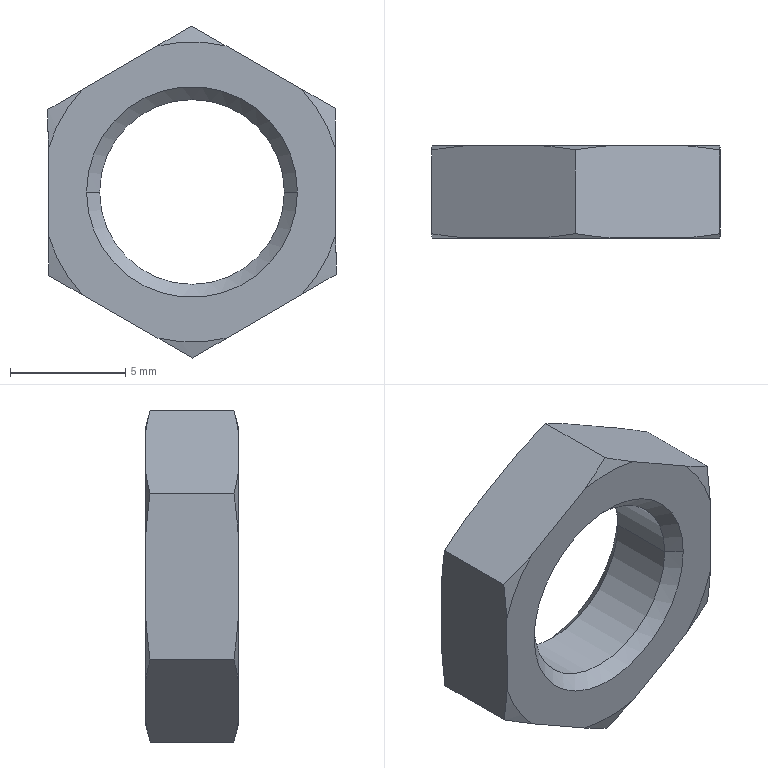Component | SolidWorks | GB_T6172.1-2000HexThinNutGradeAAndBM8-1 | 1 solid | 26 faces | box 12.48 x 4 x 14.38 mm | volume 327 mm3 | cone 16 | plane 8 | cylinder 2 | commonest cylinder face diameters 8 x2
STEP:
#1=COLOUR_RGB('',0.7922,0.8196,0.9333);
#2=FILL_AREA_STYLE_COLOUR('',#1);
#3=FILL_AREA_STYLE('',(#2));
#4=SURFACE_STYLE_FILL_AREA(#3);
#5=SURFACE_SIDE_STYLE('',(#4));
#6=SURFACE_STYLE_USAGE(.BOTH.,#5);
#7=PRESENTATION_STYLE_ASSIGNMENT((#6));
#8=CARTESIAN_POINT('',(2.795,-1.4,10.748));
#9=VERTEX_POINT('',#8);
#10=CARTESIAN_POINT('',(3.11,-1.4,10.748));
#11=VERTEX_POINT('',#10);
#12=CARTESIAN_POINT('',(2.953,-1.4,10.748));
#13=DIRECTION('',(0.,1.,0.));
#14=DIRECTION('',(-1.,0.,0.));
#15=AXIS2_PLACEMENT_3D('',#12,#13,#14);
#16=CIRCLE('',#15,0.1575);
#17=EDGE_CURVE('',#9,#11,#16,.T.);
#18=ORIENTED_EDGE('',*,*,#17,.F.);
#19=CARTESIAN_POINT('',(2.773,-1.378,10.748));
#20=VERTEX_POINT('',#19);
#21=CARTESIAN_POINT('',(2.795,-1.4,10.748));
#22=DIRECTION('',(-0.7071,0.7071,0.));
#23=VECTOR('',#22,39.37);
#24=LINE('',#21,#23);
#25=EDGE_CURVE('',#9,#20,#24,.T.);
#26=ORIENTED_EDGE('',*,*,#25,.T.);
#27=CARTESIAN_POINT('',(3.132,-1.378,10.748));
#28=VERTEX_POINT('',#27);
#29=CARTESIAN_POINT('',(2.953,-1.378,10.748));
#30=DIRECTION('',(0.,-1.,-0.));
#31=DIRECTION('',(-1.,0.,0.));
#32=AXIS2_PLACEMENT_3D('',#29,#30,#31);
#33=CIRCLE('',#32,0.1797);
#34=EDGE_CURVE('',#28,#20,#33,.T.);
#35=ORIENTED_EDGE('',*,*,#34,.F.);
#36=CARTESIAN_POINT('',(3.11,-1.4,10.748));
#37=DIRECTION('',(0.7071,0.7071,0.));
#38=VECTOR('',#37,39.37);
#39=LINE('',#36,#38);
#40=EDGE_CURVE('',#11,#28,#39,.T.);
#41=ORIENTED_EDGE('',*,*,#40,.F.);
#42=EDGE_LOOP('',(#18,#26,#35,#41));
#43=FACE_OUTER_BOUND('',#42,.T.);
#44=CARTESIAN_POINT('',(2.953,-1.4,10.748));
#45=DIRECTION('',(0.,1.,0.));
#46=DIRECTION('',(1.,0.,0.));
#47=AXIS2_PLACEMENT_3D('',#44,#45,#46);
#48=CONICAL_SURFACE('',#47,0.1575,0.7854);
#49=ADVANCED_FACE('',(#43),#48,.F.);
#50=CARTESIAN_POINT('',(3.11,-1.513,10.748));
#51=VERTEX_POINT('',#50);
#52=CARTESIAN_POINT('',(2.795,-1.513,10.748));
#53=VERTEX_POINT('',#52);
#54=CARTESIAN_POINT('',(2.953,-1.513,10.748));
#55=DIRECTION('',(0.,-1.,-0.));
#56=DIRECTION('',(-1.,0.,0.));
#57=AXIS2_PLACEMENT_3D('',#54,#55,#56);
#58=CIRCLE('',#57,0.1575);
#59=EDGE_CURVE('',#51,#53,#58,.T.);
#60=ORIENTED_EDGE('',*,*,#59,.F.);
#61=CARTESIAN_POINT('',(3.132,-1.535,10.748));
#62=VERTEX_POINT('',#61);
#63=CARTESIAN_POINT('',(3.132,-1.535,10.748));
#64=DIRECTION('',(0.7071,-0.7071,-0.));
#65=VECTOR('',#64,39.37);
#66=LINE('',#63,#65);
#67=EDGE_CURVE('',#51,#62,#66,.T.);
#68=ORIENTED_EDGE('',*,*,#67,.T.);
#69=CARTESIAN_POINT('',(2.773,-1.535,10.748));
#70=VERTEX_POINT('',#69);
#71=CARTESIAN_POINT('',(2.953,-1.535,10.748));
#72=DIRECTION('',(0.,1.,0.));
#73=DIRECTION('',(-1.,0.,0.));
#74=AXIS2_PLACEMENT_3D('',#71,#72,#73);
#75=CIRCLE('',#74,0.1797);
#76=EDGE_CURVE('',#70,#62,#75,.T.);
#77=ORIENTED_EDGE('',*,*,#76,.F.);
#78=CARTESIAN_POINT('',(2.773,-1.535,10.748));
#79=DIRECTION('',(-0.7071,-0.7071,-0.));
#80=VECTOR('',#79,39.37);
#81=LINE('',#78,#80);
#82=EDGE_CURVE('',#53,#70,#81,.T.);
#83=ORIENTED_EDGE('',*,*,#82,.F.);
#84=EDGE_LOOP('',(#60,#68,#77,#83));
#85=FACE_OUTER_BOUND('',#84,.T.);
#86=CARTESIAN_POINT('',(2.953,-1.535,10.748));
#87=DIRECTION('',(0.,-1.,-0.));
#88=DIRECTION('',(-1.,0.,0.));
#89=AXIS2_PLACEMENT_3D('',#86,#87,#88);
#90=CONICAL_SURFACE('',#89,0.1797,0.7854);
#91=ADVANCED_FACE('',(#85),#90,.F.);
#92=ORIENTED_EDGE('',*,*,#17,.T.);
#93=CARTESIAN_POINT('',(3.11,-1.378,10.748));
#94=DIRECTION('',(0.,-1.,-0.));
#95=VECTOR('',#94,39.37);
#96=LINE('',#93,#95);
#97=EDGE_CURVE('',#11,#51,#96,.T.);
#98=ORIENTED_EDGE('',*,*,#97,.T.);
#99=ORIENTED_EDGE('',*,*,#59,.T.);
#100=CARTESIAN_POINT('',(2.795,-1.378,10.748));
#101=DIRECTION('',(0.,-1.,-0.));
#102=VECTOR('',#101,39.37);
#103=LINE('',#100,#102);
#104=EDGE_CURVE('',#9,#53,#103,.T.);
#105=ORIENTED_EDGE('',*,*,#104,.F.);
#106=EDGE_LOOP('',(#92,#98,#99,#105));
#107=FACE_OUTER_BOUND('',#106,.T.);
#108=CARTESIAN_POINT('',(2.953,-1.378,10.748));
#109=DIRECTION('',(0.,-1.,-0.));
#110=DIRECTION('',(-1.,0.,0.));
#111=AXIS2_PLACEMENT_3D('',#108,#109,#110);
#112=CYLINDRICAL_SURFACE('',#111,0.1575);
#113=ADVANCED_FACE('',(#107),#112,.F.);
#114=CARTESIAN_POINT('',(2.767,-1.378,10.572));
#115=VERTEX_POINT('',#114);
#116=CARTESIAN_POINT('',(2.708,-1.385,10.606));
#117=VERTEX_POINT('',#116);
#118=CARTESIAN_POINT('',(2.767,-1.378,10.572));
#119=CARTESIAN_POINT('',(2.748,-1.38,10.583));
#120=CARTESIAN_POINT('',(2.728,-1.382,10.594));
#121=CARTESIAN_POINT('',(2.708,-1.385,10.606));
#122=B_SPLINE_CURVE_WITH_KNOTS('',3,(#118,#119,#120,#121),.UNSPECIFIED.,.F.,.F.,(4,4),(0.,0.00174),.UNSPECIFIED.);
#123=EDGE_CURVE('',#115,#117,#122,.T.);
#124=ORIENTED_EDGE('',*,*,#123,.T.);
#125=CARTESIAN_POINT('',(2.708,-1.378,10.674));
#126=VERTEX_POINT('',#125);
#127=CARTESIAN_POINT('',(2.708,-1.385,10.606));
#128=CARTESIAN_POINT('',(2.708,-1.382,10.628));
#129=CARTESIAN_POINT('',(2.708,-1.38,10.651));
#130=CARTESIAN_POINT('',(2.708,-1.378,10.674));
#131=B_SPLINE_CURVE_WITH_KNOTS('',3,(#127,#128,#129,#130),.UNSPECIFIED.,.F.,.F.,(4,4),(0.005002,0.006741),.UNSPECIFIED.);
#132=EDGE_CURVE('',#117,#126,#131,.T.);
#133=ORIENTED_EDGE('',*,*,#132,.T.);
#134=CARTESIAN_POINT('',(2.953,-1.378,10.748));
#135=DIRECTION('',(0.,-1.,-0.));
#136=DIRECTION('',(-1.,0.,0.));
#137=AXIS2_PLACEMENT_3D('',#134,#135,#136);
#138=CIRCLE('',#137,0.2559);
#139=EDGE_CURVE('',#126,#115,#138,.T.);
#140=ORIENTED_EDGE('',*,*,#139,.T.);
#141=EDGE_LOOP('',(#124,#133,#140));
#142=FACE_OUTER_BOUND('',#141,.T.);
#143=CARTESIAN_POINT('',(2.953,-1.378,10.748));
#144=DIRECTION('',(0.,-1.,-0.));
#145=DIRECTION('',(1.,0.,0.));
#146=AXIS2_PLACEMENT_3D('',#143,#144,#145);
#147=CONICAL_SURFACE('',#146,0.2559,1.309);
#148=ADVANCED_FACE('',(#142),#147,.T.);
#149=CARTESIAN_POINT('',(3.013,-1.378,10.499));
#150=VERTEX_POINT('',#149);
#151=CARTESIAN_POINT('',(2.954,-1.385,10.465));
#152=VERTEX_POINT('',#151);
#153=CARTESIAN_POINT('',(3.013,-1.378,10.499));
#154=CARTESIAN_POINT('',(2.993,-1.38,10.488));
#155=CARTESIAN_POINT('',(2.973,-1.382,10.476));
#156=CARTESIAN_POINT('',(2.954,-1.385,10.465));
#157=B_SPLINE_CURVE_WITH_KNOTS('',3,(#153,#154,#155,#156),.UNSPECIFIED.,.F.,.F.,(4,4),(0.,0.00174),.UNSPECIFIED.);
#158=EDGE_CURVE('',#150,#152,#157,.T.);
#159=ORIENTED_EDGE('',*,*,#158,.T.);
#160=CARTESIAN_POINT('',(2.895,-1.378,10.499));
#161=VERTEX_POINT('',#160);
#162=CARTESIAN_POINT('',(2.954,-1.385,10.465));
#163=CARTESIAN_POINT('',(2.934,-1.382,10.476));
#164=CARTESIAN_POINT('',(2.915,-1.38,10.487));
#165=CARTESIAN_POINT('',(2.895,-1.378,10.499));
#166=B_SPLINE_CURVE_WITH_KNOTS('',3,(#162,#163,#164,#165),.UNSPECIFIED.,.F.,.F.,(4,4),(0.00577,0.00751),.UNSPECIFIED.);
#167=EDGE_CURVE('',#152,#161,#166,.T.);
#168=ORIENTED_EDGE('',*,*,#167,.T.);
#169=CARTESIAN_POINT('',(2.953,-1.378,10.748));
#170=DIRECTION('',(0.,-1.,-0.));
#171=DIRECTION('',(-1.,0.,0.));
#172=AXIS2_PLACEMENT_3D('',#169,#170,#171);
#173=CIRCLE('',#172,0.2559);
#174=EDGE_CURVE('',#161,#150,#173,.T.);
#175=ORIENTED_EDGE('',*,*,#174,.T.);
#176=EDGE_LOOP('',(#159,#168,#175));
#177=FACE_OUTER_BOUND('',#176,.T.);
#178=CARTESIAN_POINT('',(2.953,-1.378,10.748));
#179=DIRECTION('',(0.,-1.,-0.));
#180=DIRECTION('',(1.,0.,0.));
#181=AXIS2_PLACEMENT_3D('',#178,#179,#180);
#182=CONICAL_SURFACE('',#181,0.2559,1.309);
#183=ADVANCED_FACE('',(#177),#182,.T.);
#184=CARTESIAN_POINT('',(3.198,-1.385,10.607));
#185=VERTEX_POINT('',#184);
#186=CARTESIAN_POINT('',(3.14,-1.378,10.573));
#187=VERTEX_POINT('',#186);
#188=CARTESIAN_POINT('',(3.198,-1.385,10.607));
#189=CARTESIAN_POINT('',(3.179,-1.382,10.596));
#190=CARTESIAN_POINT('',(3.159,-1.38,10.585));
#191=CARTESIAN_POINT('',(3.14,-1.378,10.573));
#192=B_SPLINE_CURVE_WITH_KNOTS('',3,(#188,#189,#190,#191),.UNSPECIFIED.,.F.,.F.,(4,4),(0.005796,0.007536),.UNSPECIFIED.);
#193=EDGE_CURVE('',#185,#187,#192,.T.);
#194=ORIENTED_EDGE('',*,*,#193,.T.);
#195=CARTESIAN_POINT('',(3.198,-1.378,10.676));
#196=VERTEX_POINT('',#195);
#197=CARTESIAN_POINT('',(2.953,-1.378,10.748));
#198=DIRECTION('',(0.,1.,0.));
#199=DIRECTION('',(1.,0.,0.));
#200=AXIS2_PLACEMENT_3D('',#197,#198,#199);
#201=CIRCLE('',#200,0.2559);
#202=EDGE_CURVE('',#196,#187,#201,.T.);
#203=ORIENTED_EDGE('',*,*,#202,.F.);
#204=CARTESIAN_POINT('',(3.198,-1.378,10.676));
#205=CARTESIAN_POINT('',(3.198,-1.38,10.653));
#206=CARTESIAN_POINT('',(3.198,-1.382,10.63));
#207=CARTESIAN_POINT('',(3.198,-1.385,10.607));
#208=B_SPLINE_CURVE_WITH_KNOTS('',3,(#204,#205,#206,#207),.UNSPECIFIED.,.F.,.F.,(4,4),(0.,0.00174),.UNSPECIFIED.);
#209=EDGE_CURVE('',#196,#185,#208,.T.);
#210=ORIENTED_EDGE('',*,*,#209,.T.);
#211=EDGE_LOOP('',(#194,#203,#210));
#212=FACE_OUTER_BOUND('',#211,.T.);
#213=CARTESIAN_POINT('',(2.953,-1.378,10.748));
#214=DIRECTION('',(0.,-1.,-0.));
#215=DIRECTION('',(1.,0.,0.));
#216=AXIS2_PLACEMENT_3D('',#213,#214,#215);
#217=CONICAL_SURFACE('',#216,0.2559,1.309);
#218=ADVANCED_FACE('',(#212),#217,.T.);
#219=CARTESIAN_POINT('',(3.138,-1.378,10.924));
#220=VERTEX_POINT('',#219);
#221=CARTESIAN_POINT('',(3.197,-1.385,10.891));
#222=VERTEX_POINT('',#221);
#223=CARTESIAN_POINT('',(3.138,-1.378,10.924));
#224=CARTESIAN_POINT('',(3.158,-1.38,10.913));
#225=CARTESIAN_POINT('',(3.178,-1.382,10.902));
#226=CARTESIAN_POINT('',(3.197,-1.385,10.891));
#227=B_SPLINE_CURVE_WITH_KNOTS('',3,(#223,#224,#225,#226),.UNSPECIFIED.,.F.,.F.,(4,4),(0.,0.00174),.UNSPECIFIED.);
#228=EDGE_CURVE('',#220,#222,#227,.T.);
#229=ORIENTED_EDGE('',*,*,#228,.T.);
#230=CARTESIAN_POINT('',(3.198,-1.378,10.822));
#231=VERTEX_POINT('',#230);
#232=CARTESIAN_POINT('',(3.197,-1.385,10.891));
#233=CARTESIAN_POINT('',(3.197,-1.382,10.868));
#234=CARTESIAN_POINT('',(3.198,-1.38,10.845));
#235=CARTESIAN_POINT('',(3.198,-1.378,10.822));
#236=B_SPLINE_CURVE_WITH_KNOTS('',3,(#232,#233,#234,#235),.UNSPECIFIED.,.F.,.F.,(4,4),(0.005002,0.006741),.UNSPECIFIED.);
#237=EDGE_CURVE('',#222,#231,#236,.T.);
#238=ORIENTED_EDGE('',*,*,#237,.T.);
#239=CARTESIAN_POINT('',(2.953,-1.378,10.748));
#240=DIRECTION('',(0.,-1.,-0.));
#241=DIRECTION('',(-1.,0.,0.));
#242=AXIS2_PLACEMENT_3D('',#239,#240,#241);
#243=CIRCLE('',#242,0.2559);
#244=EDGE_CURVE('',#231,#220,#243,.T.);
#245=ORIENTED_EDGE('',*,*,#244,.T.);
#246=EDGE_LOOP('',(#229,#238,#245));
#247=FACE_OUTER_BOUND('',#246,.T.);
#248=CARTESIAN_POINT('',(2.953,-1.378,10.748));
#249=DIRECTION('',(0.,-1.,-0.));
#250=DIRECTION('',(1.,0.,0.));
#251=AXIS2_PLACEMENT_3D('',#248,#249,#250);
#252=CONICAL_SURFACE('',#251,0.2559,1.309);
#253=ADVANCED_FACE('',(#247),#252,.T.);
#254=CARTESIAN_POINT('',(2.893,-1.378,10.997));
#255=VERTEX_POINT('',#254);
#256=CARTESIAN_POINT('',(2.952,-1.385,11.031));
#257=VERTEX_POINT('',#256);
#258=CARTESIAN_POINT('',(2.893,-1.378,10.997));
#259=CARTESIAN_POINT('',(2.912,-1.38,11.008));
#260=CARTESIAN_POINT('',(2.932,-1.382,11.02));
#261=CARTESIAN_POINT('',(2.952,-1.385,11.031));
#262=B_SPLINE_CURVE_WITH_KNOTS('',3,(#258,#259,#260,#261),.UNSPECIFIED.,.F.,.F.,(4,4),(0.,0.00174),.UNSPECIFIED.);
#263=EDGE_CURVE('',#255,#257,#262,.T.);
#264=ORIENTED_EDGE('',*,*,#263,.T.);
#265=CARTESIAN_POINT('',(3.011,-1.378,10.997));
#266=VERTEX_POINT('',#265);
#267=CARTESIAN_POINT('',(2.952,-1.385,11.031));
#268=CARTESIAN_POINT('',(2.971,-1.382,11.02));
#269=CARTESIAN_POINT('',(2.991,-1.38,11.009));
#270=CARTESIAN_POINT('',(3.011,-1.378,10.997));
#271=B_SPLINE_CURVE_WITH_KNOTS('',3,(#267,#268,#269,#270),.UNSPECIFIED.,.F.,.F.,(4,4),(0.00577,0.00751),.UNSPECIFIED.);
#272=EDGE_CURVE('',#257,#266,#271,.T.);
#273=ORIENTED_EDGE('',*,*,#272,.T.);
#274=CARTESIAN_POINT('',(2.953,-1.378,10.748));
#275=DIRECTION('',(0.,-1.,-0.));
#276=DIRECTION('',(-1.,0.,0.));
#277=AXIS2_PLACEMENT_3D('',#274,#275,#276);
#278=CIRCLE('',#277,0.2559);
#279=EDGE_CURVE('',#266,#255,#278,.T.);
#280=ORIENTED_EDGE('',*,*,#279,.T.);
#281=EDGE_LOOP('',(#264,#273,#280));
#282=FACE_OUTER_BOUND('',#281,.T.);
#283=CARTESIAN_POINT('',(2.953,-1.378,10.748));
#284=DIRECTION('',(0.,-1.,-0.));
#285=DIRECTION('',(1.,0.,0.));
#286=AXIS2_PLACEMENT_3D('',#283,#284,#285);
#287=CONICAL_SURFACE('',#286,0.2559,1.309);
#288=ADVANCED_FACE('',(#282),#287,.T.);
#289=CARTESIAN_POINT('',(2.707,-1.378,10.82));
#290=VERTEX_POINT('',#289);
#291=CARTESIAN_POINT('',(2.707,-1.385,10.889));
#292=VERTEX_POINT('',#291);
#293=CARTESIAN_POINT('',(2.707,-1.378,10.82));
#294=CARTESIAN_POINT('',(2.707,-1.38,10.843));
#295=CARTESIAN_POINT('',(2.707,-1.382,10.866));
#296=CARTESIAN_POINT('',(2.707,-1.385,10.889));
#297=B_SPLINE_CURVE_WITH_KNOTS('',3,(#293,#294,#295,#296),.UNSPECIFIED.,.F.,.F.,(4,4),(0.,0.00174),.UNSPECIFIED.);
#298=EDGE_CURVE('',#290,#292,#297,.T.);
#299=ORIENTED_EDGE('',*,*,#298,.T.);
#300=CARTESIAN_POINT('',(2.766,-1.378,10.923));
#301=VERTEX_POINT('',#300);
#302=CARTESIAN_POINT('',(2.707,-1.385,10.889));
#303=CARTESIAN_POINT('',(2.727,-1.382,10.9));
#304=CARTESIAN_POINT('',(2.746,-1.38,10.911));
#305=CARTESIAN_POINT('',(2.766,-1.378,10.923));
#306=B_SPLINE_CURVE_WITH_KNOTS('',3,(#302,#303,#304,#305),.UNSPECIFIED.,.F.,.F.,(4,4),(0.005796,0.007536),.UNSPECIFIED.);
#307=EDGE_CURVE('',#292,#301,#306,.T.);
#308=ORIENTED_EDGE('',*,*,#307,.T.);
#309=CARTESIAN_POINT('',(2.953,-1.378,10.748));
#310=DIRECTION('',(0.,-1.,-0.));
#311=DIRECTION('',(-1.,0.,0.));
#312=AXIS2_PLACEMENT_3D('',#309,#310,#311);
#313=CIRCLE('',#312,0.2559);
#314=EDGE_CURVE('',#301,#290,#313,.T.);
#315=ORIENTED_EDGE('',*,*,#314,.T.);
#316=EDGE_LOOP('',(#299,#308,#315));
#317=FACE_OUTER_BOUND('',#316,.T.);
#318=CARTESIAN_POINT('',(2.953,-1.378,10.748));
#319=DIRECTION('',(0.,-1.,-0.));
#320=DIRECTION('',(1.,0.,0.));
#321=AXIS2_PLACEMENT_3D('',#318,#319,#320);
#322=CONICAL_SURFACE('',#321,0.2559,1.309);
#323=ADVANCED_FACE('',(#317),#322,.T.);
#324=CARTESIAN_POINT('',(2.954,-1.528,10.465));
#325=VERTEX_POINT('',#324);
#326=CARTESIAN_POINT('',(3.013,-1.535,10.499));
#327=VERTEX_POINT('',#326);
#328=CARTESIAN_POINT('',(2.954,-1.528,10.465));
#329=CARTESIAN_POINT('',(2.973,-1.531,10.476));
#330=CARTESIAN_POINT('',(2.993,-1.534,10.488));
#331=CARTESIAN_POINT('',(3.013,-1.535,10.499));
#332=B_SPLINE_CURVE_WITH_KNOTS('',3,(#328,#329,#330,#331),.UNSPECIFIED.,.F.,.F.,(4,4),(0.005796,0.007536),.UNSPECIFIED.);
#333=EDGE_CURVE('',#325,#327,#332,.T.);
#334=ORIENTED_EDGE('',*,*,#333,.T.);
#335=CARTESIAN_POINT('',(2.895,-1.535,10.499));
#336=VERTEX_POINT('',#335);
#337=CARTESIAN_POINT('',(2.953,-1.535,10.748));
#338=DIRECTION('',(0.,-1.,-0.));
#339=DIRECTION('',(-1.,0.,0.));
#340=AXIS2_PLACEMENT_3D('',#337,#338,#339);
#341=CIRCLE('',#340,0.2559);
#342=EDGE_CURVE('',#336,#327,#341,.T.);
#343=ORIENTED_EDGE('',*,*,#342,.F.);
#344=CARTESIAN_POINT('',(2.895,-1.535,10.499));
#345=CARTESIAN_POINT('',(2.915,-1.534,10.487));
#346=CARTESIAN_POINT('',(2.934,-1.531,10.476));
#347=CARTESIAN_POINT('',(2.954,-1.528,10.465));
#348=B_SPLINE_CURVE_WITH_KNOTS('',3,(#344,#345,#346,#347),.UNSPECIFIED.,.F.,.F.,(4,4),(0.,0.00174),.UNSPECIFIED.);
#349=EDGE_CURVE('',#336,#325,#348,.T.);
#350=ORIENTED_EDGE('',*,*,#349,.T.);
#351=EDGE_LOOP('',(#334,#343,#350));
#352=FACE_OUTER_BOUND('',#351,.T.);
#353=CARTESIAN_POINT('',(2.953,-1.535,10.748));
#354=DIRECTION('',(0.,1.,0.));
#355=DIRECTION('',(-1.,0.,0.));
#356=AXIS2_PLACEMENT_3D('',#353,#354,#355);
#357=CONICAL_SURFACE('',#356,0.2559,1.309);
#358=ADVANCED_FACE('',(#352),#357,.T.);
#359=CARTESIAN_POINT('',(2.708,-1.528,10.606));
#360=VERTEX_POINT('',#359);
#361=CARTESIAN_POINT('',(2.767,-1.535,10.572));
#362=VERTEX_POINT('',#361);
#363=CARTESIAN_POINT('',(2.708,-1.528,10.606));
#364=CARTESIAN_POINT('',(2.728,-1.531,10.594));
#365=CARTESIAN_POINT('',(2.748,-1.534,10.583));
#366=CARTESIAN_POINT('',(2.767,-1.535,10.572));
#367=B_SPLINE_CURVE_WITH_KNOTS('',3,(#363,#364,#365,#366),.UNSPECIFIED.,.F.,.F.,(4,4),(0.00577,0.00751),.UNSPECIFIED.);
#368=EDGE_CURVE('',#360,#362,#367,.T.);
#369=ORIENTED_EDGE('',*,*,#368,.T.);
#370=CARTESIAN_POINT('',(2.708,-1.535,10.674));
#371=VERTEX_POINT('',#370);
#372=CARTESIAN_POINT('',(2.953,-1.535,10.748));
#373=DIRECTION('',(0.,-1.,-0.));
#374=DIRECTION('',(-1.,0.,0.));
#375=AXIS2_PLACEMENT_3D('',#372,#373,#374);
#376=CIRCLE('',#375,0.2559);
#377=EDGE_CURVE('',#371,#362,#376,.T.);
#378=ORIENTED_EDGE('',*,*,#377,.F.);
#379=CARTESIAN_POINT('',(2.708,-1.535,10.674));
#380=CARTESIAN_POINT('',(2.708,-1.534,10.651));
#381=CARTESIAN_POINT('',(2.708,-1.531,10.628));
#382=CARTESIAN_POINT('',(2.708,-1.528,10.606));
#383=B_SPLINE_CURVE_WITH_KNOTS('',3,(#379,#380,#381,#382),.UNSPECIFIED.,.F.,.F.,(4,4),(0.,0.00174),.UNSPECIFIED.);
#384=EDGE_CURVE('',#371,#360,#383,.T.);
#385=ORIENTED_EDGE('',*,*,#384,.T.);
#386=EDGE_LOOP('',(#369,#378,#385));
#387=FACE_OUTER_BOUND('',#386,.T.);
#388=CARTESIAN_POINT('',(2.953,-1.535,10.748));
#389=DIRECTION('',(0.,1.,0.));
#390=DIRECTION('',(-1.,0.,0.));
#391=AXIS2_PLACEMENT_3D('',#388,#389,#390);
#392=CONICAL_SURFACE('',#391,0.2559,1.309);
#393=ADVANCED_FACE('',(#387),#392,.T.);
#394=CARTESIAN_POINT('',(2.707,-1.528,10.889));
#395=VERTEX_POINT('',#394);
#396=CARTESIAN_POINT('',(2.707,-1.535,10.82));
#397=VERTEX_POINT('',#396);
#398=CARTESIAN_POINT('',(2.707,-1.528,10.889));
#399=CARTESIAN_POINT('',(2.707,-1.531,10.866));
#400=CARTESIAN_POINT('',(2.707,-1.534,10.843));
#401=CARTESIAN_POINT('',(2.707,-1.535,10.82));
#402=B_SPLINE_CURVE_WITH_KNOTS('',3,(#398,#399,#400,#401),.UNSPECIFIED.,.F.,.F.,(4,4),(0.005002,0.006741),.UNSPECIFIED.);
#403=EDGE_CURVE('',#395,#397,#402,.T.);
#404=ORIENTED_EDGE('',*,*,#403,.T.);
#405=CARTESIAN_POINT('',(2.766,-1.535,10.923));
#406=VERTEX_POINT('',#405);
#407=CARTESIAN_POINT('',(2.953,-1.535,10.748));
#408=DIRECTION('',(0.,-1.,-0.));
#409=DIRECTION('',(-1.,0.,0.));
#410=AXIS2_PLACEMENT_3D('',#407,#408,#409);
#411=CIRCLE('',#410,0.2559);
#412=EDGE_CURVE('',#406,#397,#411,.T.);
#413=ORIENTED_EDGE('',*,*,#412,.F.);
#414=CARTESIAN_POINT('',(2.766,-1.535,10.923));
#415=CARTESIAN_POINT('',(2.746,-1.534,10.911));
#416=CARTESIAN_POINT('',(2.727,-1.531,10.9));
#417=CARTESIAN_POINT('',(2.707,-1.528,10.889));
#418=B_SPLINE_CURVE_WITH_KNOTS('',3,(#414,#415,#416,#417),.UNSPECIFIED.,.F.,.F.,(4,4),(0.,0.00174),.UNSPECIFIED.);
#419=EDGE_CURVE('',#406,#395,#418,.T.);
#420=ORIENTED_EDGE('',*,*,#419,.T.);
#421=EDGE_LOOP('',(#404,#413,#420));
#422=FACE_OUTER_BOUND('',#421,.T.);
#423=CARTESIAN_POINT('',(2.953,-1.535,10.748));
#424=DIRECTION('',(0.,1.,0.));
#425=DIRECTION('',(-1.,0.,0.));
#426=AXIS2_PLACEMENT_3D('',#423,#424,#425);
#427=CONICAL_SURFACE('',#426,0.2559,1.309);
#428=ADVANCED_FACE('',(#422),#427,.T.);
#429=CARTESIAN_POINT('',(2.952,-1.528,11.031));
#430=VERTEX_POINT('',#429);
#431=CARTESIAN_POINT('',(2.893,-1.535,10.997));
#432=VERTEX_POINT('',#431);
#433=CARTESIAN_POINT('',(2.952,-1.528,11.031));
#434=CARTESIAN_POINT('',(2.932,-1.531,11.02));
#435=CARTESIAN_POINT('',(2.912,-1.534,11.008));
#436=CARTESIAN_POINT('',(2.893,-1.535,10.997));
#437=B_SPLINE_CURVE_WITH_KNOTS('',3,(#433,#434,#435,#436),.UNSPECIFIED.,.F.,.F.,(4,4),(0.005796,0.007536),.UNSPECIFIED.);
#438=EDGE_CURVE('',#430,#432,#437,.T.);
#439=ORIENTED_EDGE('',*,*,#438,.T.);
#440=CARTESIAN_POINT('',(3.011,-1.535,10.997));
#441=VERTEX_POINT('',#440);
#442=CARTESIAN_POINT('',(2.953,-1.535,10.748));
#443=DIRECTION('',(0.,-1.,-0.));
#444=DIRECTION('',(-1.,0.,0.));
#445=AXIS2_PLACEMENT_3D('',#442,#443,#444);
#446=CIRCLE('',#445,0.2559);
#447=EDGE_CURVE('',#441,#432,#446,.T.);
#448=ORIENTED_EDGE('',*,*,#447,.F.);
#449=CARTESIAN_POINT('',(3.011,-1.535,10.997));
#450=CARTESIAN_POINT('',(2.991,-1.534,11.009));
#451=CARTESIAN_POINT('',(2.971,-1.531,11.02));
#452=CARTESIAN_POINT('',(2.952,-1.528,11.031));
#453=B_SPLINE_CURVE_WITH_KNOTS('',3,(#449,#450,#451,#452),.UNSPECIFIED.,.F.,.F.,(4,4),(0.,0.00174),.UNSPECIFIED.);
#454=EDGE_CURVE('',#441,#430,#453,.T.);
#455=ORIENTED_EDGE('',*,*,#454,.T.);
#456=EDGE_LOOP('',(#439,#448,#455));
#457=FACE_OUTER_BOUND('',#456,.T.);
#458=CARTESIAN_POINT('',(2.953,-1.535,10.748));
#459=DIRECTION('',(0.,1.,0.));
#460=DIRECTION('',(-1.,0.,0.));
#461=AXIS2_PLACEMENT_3D('',#458,#459,#460);
#462=CONICAL_SURFACE('',#461,0.2559,1.309);
#463=ADVANCED_FACE('',(#457),#462,.T.);
#464=CARTESIAN_POINT('',(3.14,-1.535,10.573));
#465=VERTEX_POINT('',#464);
#466=CARTESIAN_POINT('',(3.198,-1.528,10.607));
#467=VERTEX_POINT('',#466);
#468=CARTESIAN_POINT('',(3.14,-1.535,10.573));
#469=CARTESIAN_POINT('',(3.159,-1.534,10.585));
#470=CARTESIAN_POINT('',(3.179,-1.531,10.596));
#471=CARTESIAN_POINT('',(3.198,-1.528,10.607));
#472=B_SPLINE_CURVE_WITH_KNOTS('',3,(#468,#469,#470,#471),.UNSPECIFIED.,.F.,.F.,(4,4),(0.,0.00174),.UNSPECIFIED.);
#473=EDGE_CURVE('',#465,#467,#472,.T.);
#474=ORIENTED_EDGE('',*,*,#473,.T.);
#475=CARTESIAN_POINT('',(3.198,-1.535,10.676));
#476=VERTEX_POINT('',#475);
#477=CARTESIAN_POINT('',(3.198,-1.528,10.607));
#478=CARTESIAN_POINT('',(3.198,-1.531,10.63));
#479=CARTESIAN_POINT('',(3.198,-1.534,10.653));
#480=CARTESIAN_POINT('',(3.198,-1.535,10.676));
#481=B_SPLINE_CURVE_WITH_KNOTS('',3,(#477,#478,#479,#480),.UNSPECIFIED.,.F.,.F.,(4,4),(0.005002,0.006741),.UNSPECIFIED.);
#482=EDGE_CURVE('',#467,#476,#481,.T.);
#483=ORIENTED_EDGE('',*,*,#482,.T.);
#484=CARTESIAN_POINT('',(2.953,-1.535,10.748));
#485=DIRECTION('',(0.,-1.,-0.));
#486=DIRECTION('',(-1.,0.,0.));
#487=AXIS2_PLACEMENT_3D('',#484,#485,#486);
#488=CIRCLE('',#487,0.2559);
#489=EDGE_CURVE('',#465,#476,#488,.T.);
#490=ORIENTED_EDGE('',*,*,#489,.F.);
#491=EDGE_LOOP('',(#474,#483,#490));
#492=FACE_OUTER_BOUND('',#491,.T.);
#493=CARTESIAN_POINT('',(2.953,-1.535,10.748));
#494=DIRECTION('',(0.,1.,0.));
#495=DIRECTION('',(-1.,0.,0.));
#496=AXIS2_PLACEMENT_3D('',#493,#494,#495);
#497=CONICAL_SURFACE('',#496,0.2559,1.309);
#498=ADVANCED_FACE('',(#492),#497,.T.);
#499=CARTESIAN_POINT('',(3.197,-1.528,10.891));
#500=VERTEX_POINT('',#499);
#501=CARTESIAN_POINT('',(3.138,-1.535,10.924));
#502=VERTEX_POINT('',#501);
#503=CARTESIAN_POINT('',(3.197,-1.528,10.891));
#504=CARTESIAN_POINT('',(3.178,-1.531,10.902));
#505=CARTESIAN_POINT('',(3.158,-1.534,10.913));
#506=CARTESIAN_POINT('',(3.138,-1.535,10.924));
#507=B_SPLINE_CURVE_WITH_KNOTS('',3,(#503,#504,#505,#506),.UNSPECIFIED.,.F.,.F.,(4,4),(0.00577,0.00751),.UNSPECIFIED.);
#508=EDGE_CURVE('',#500,#502,#507,.T.);
#509=ORIENTED_EDGE('',*,*,#508,.T.);
#510=CARTESIAN_POINT('',(3.198,-1.535,10.822));
#511=VERTEX_POINT('',#510);
#512=CARTESIAN_POINT('',(2.953,-1.535,10.748));
#513=DIRECTION('',(0.,-1.,-0.));
#514=DIRECTION('',(-1.,0.,0.));
#515=AXIS2_PLACEMENT_3D('',#512,#513,#514);
#516=CIRCLE('',#515,0.2559);
#517=EDGE_CURVE('',#511,#502,#516,.T.);
#518=ORIENTED_EDGE('',*,*,#517,.F.);
#519=CARTESIAN_POINT('',(3.198,-1.535,10.822));
#520=CARTESIAN_POINT('',(3.198,-1.534,10.845));
#521=CARTESIAN_POINT('',(3.197,-1.531,10.868));
#522=CARTESIAN_POINT('',(3.197,-1.528,10.891));
#523=B_SPLINE_CURVE_WITH_KNOTS('',3,(#519,#520,#521,#522),.UNSPECIFIED.,.F.,.F.,(4,4),(0.,0.00174),.UNSPECIFIED.);
#524=EDGE_CURVE('',#511,#500,#523,.T.);
#525=ORIENTED_EDGE('',*,*,#524,.T.);
#526=EDGE_LOOP('',(#509,#518,#525));
#527=FACE_OUTER_BOUND('',#526,.T.);
#528=CARTESIAN_POINT('',(2.953,-1.535,10.748));
#529=DIRECTION('',(0.,1.,0.));
#530=DIRECTION('',(-1.,0.,0.));
#531=AXIS2_PLACEMENT_3D('',#528,#529,#530);
#532=CONICAL_SURFACE('',#531,0.2559,1.309);
#533=ADVANCED_FACE('',(#527),#532,.T.);
#534=ORIENTED_EDGE('',*,*,#76,.T.);
#535=CARTESIAN_POINT('',(2.953,-1.535,10.748));
#536=DIRECTION('',(0.,1.,0.));
#537=DIRECTION('',(-1.,0.,0.));
#538=AXIS2_PLACEMENT_3D('',#535,#536,#537);
#539=CIRCLE('',#538,0.1797);
#540=EDGE_CURVE('',#62,#70,#539,.T.);
#541=ORIENTED_EDGE('',*,*,#540,.T.);
#542=EDGE_LOOP('',(#534,#541));
#543=FACE_BOUND('',#542,.T.);
#544=CARTESIAN_POINT('',(2.708,-1.535,10.606));
#545=DIRECTION('',(-0.003934,-0.,1.));
#546=VECTOR('',#545,39.37);
#547=LINE('',#544,#546);
#548=EDGE_CURVE('',#371,#397,#547,.T.);
#549=ORIENTED_EDGE('',*,*,#548,.F.);
#550=ORIENTED_EDGE('',*,*,#377,.T.);
#551=CARTESIAN_POINT('',(2.954,-1.535,10.465));
#552=DIRECTION('',(-0.868,-0.,0.4966));
#553=VECTOR('',#552,39.37);
#554=LINE('',#551,#553);
#555=EDGE_CURVE('',#336,#362,#554,.T.);
#556=ORIENTED_EDGE('',*,*,#555,.F.);
#557=ORIENTED_EDGE('',*,*,#342,.T.);
#558=CARTESIAN_POINT('',(3.198,-1.535,10.607));
#559=DIRECTION('',(-0.8641,0.,-0.5034));
#560=VECTOR('',#559,39.37);
#561=LINE('',#558,#560);
#562=EDGE_CURVE('',#465,#327,#561,.T.);
#563=ORIENTED_EDGE('',*,*,#562,.F.);
#564=ORIENTED_EDGE('',*,*,#489,.T.);
#565=CARTESIAN_POINT('',(3.197,-1.535,10.891));
#566=DIRECTION('',(0.003934,0.,-1.));
#567=VECTOR('',#566,39.37);
#568=LINE('',#565,#567);
#569=EDGE_CURVE('',#511,#476,#568,.T.);
#570=ORIENTED_EDGE('',*,*,#569,.F.);
#571=ORIENTED_EDGE('',*,*,#517,.T.);
#572=CARTESIAN_POINT('',(2.952,-1.535,11.031));
#573=DIRECTION('',(0.868,0.,-0.4966));
#574=VECTOR('',#573,39.37);
#575=LINE('',#572,#574);
#576=EDGE_CURVE('',#441,#502,#575,.T.);
#577=ORIENTED_EDGE('',*,*,#576,.F.);
#578=ORIENTED_EDGE('',*,*,#447,.T.);
#579=CARTESIAN_POINT('',(2.707,-1.535,10.889));
#580=DIRECTION('',(0.8641,-0.,0.5034));
#581=VECTOR('',#580,39.37);
#582=LINE('',#579,#581);
#583=EDGE_CURVE('',#406,#432,#582,.T.);
#584=ORIENTED_EDGE('',*,*,#583,.F.);
#585=ORIENTED_EDGE('',*,*,#412,.T.);
#586=EDGE_LOOP('',(#549,#550,#556,#557,#563,#564,#570,#571,#577,#578,#584,#585));
#587=FACE_OUTER_BOUND('',#586,.T.);
#588=CARTESIAN_POINT('',(3.443,-1.535,10.75));
#589=DIRECTION('',(0.,-1.,-0.));
#590=DIRECTION('',(0.,-0.,1.));
#591=AXIS2_PLACEMENT_3D('',#588,#589,#590);
#592=PLANE('',#591);
#593=ADVANCED_FACE('',(#543,#587),#592,.T.);
#594=ORIENTED_EDGE('',*,*,#34,.T.);
#595=CARTESIAN_POINT('',(2.953,-1.378,10.748));
#596=DIRECTION('',(0.,-1.,-0.));
#597=DIRECTION('',(-1.,0.,0.));
#598=AXIS2_PLACEMENT_3D('',#595,#596,#597);
#599=CIRCLE('',#598,0.1797);
#600=EDGE_CURVE('',#20,#28,#599,.T.);
#601=ORIENTED_EDGE('',*,*,#600,.T.);
#602=EDGE_LOOP('',(#594,#601));
#603=FACE_BOUND('',#602,.T.);
#604=ORIENTED_EDGE('',*,*,#139,.F.);
#605=CARTESIAN_POINT('',(2.708,-1.378,10.606));
#606=DIRECTION('',(-0.003934,-0.,1.));
#607=VECTOR('',#606,39.37);
#608=LINE('',#605,#607);
#609=EDGE_CURVE('',#126,#290,#608,.T.);
#610=ORIENTED_EDGE('',*,*,#609,.T.);
#611=ORIENTED_EDGE('',*,*,#314,.F.);
#612=CARTESIAN_POINT('',(2.707,-1.378,10.889));
#613=DIRECTION('',(0.8641,-0.,0.5034));
#614=VECTOR('',#613,39.37);
#615=LINE('',#612,#614);
#616=EDGE_CURVE('',#301,#255,#615,.T.);
#617=ORIENTED_EDGE('',*,*,#616,.T.);
#618=ORIENTED_EDGE('',*,*,#279,.F.);
#619=CARTESIAN_POINT('',(2.952,-1.378,11.031));
#620=DIRECTION('',(0.868,0.,-0.4966));
#621=VECTOR('',#620,39.37);
#622=LINE('',#619,#621);
#623=EDGE_CURVE('',#266,#220,#622,.T.);
#624=ORIENTED_EDGE('',*,*,#623,.T.);
#625=ORIENTED_EDGE('',*,*,#244,.F.);
#626=CARTESIAN_POINT('',(3.197,-1.378,10.891));
#627=DIRECTION('',(0.003934,0.,-1.));
#628=VECTOR('',#627,39.37);
#629=LINE('',#626,#628);
#630=EDGE_CURVE('',#231,#196,#629,.T.);
#631=ORIENTED_EDGE('',*,*,#630,.T.);
#632=ORIENTED_EDGE('',*,*,#202,.T.);
#633=CARTESIAN_POINT('',(3.198,-1.378,10.607));
#634=DIRECTION('',(-0.8641,0.,-0.5034));
#635=VECTOR('',#634,39.37);
#636=LINE('',#633,#635);
#637=EDGE_CURVE('',#187,#150,#636,.T.);
#638=ORIENTED_EDGE('',*,*,#637,.T.);
#639=ORIENTED_EDGE('',*,*,#174,.F.);
#640=CARTESIAN_POINT('',(2.954,-1.378,10.465));
#641=DIRECTION('',(-0.868,-0.,0.4966));
#642=VECTOR('',#641,39.37);
#643=LINE('',#640,#642);
#644=EDGE_CURVE('',#161,#115,#643,.T.);
#645=ORIENTED_EDGE('',*,*,#644,.T.);
#646=EDGE_LOOP('',(#604,#610,#611,#617,#618,#624,#625,#631,#632,#638,#639,#645));
#647=FACE_OUTER_BOUND('',#646,.T.);
#648=CARTESIAN_POINT('',(3.443,-1.378,10.75));
#649=DIRECTION('',(0.,-1.,-0.));
#650=DIRECTION('',(0.,-0.,1.));
#651=AXIS2_PLACEMENT_3D('',#648,#649,#650);
#652=PLANE('',#651);
#653=ADVANCED_FACE('',(#603,#647),#652,.F.);
#654=ORIENTED_EDGE('',*,*,#237,.F.);
#655=CARTESIAN_POINT('',(3.197,-1.378,10.891));
#656=DIRECTION('',(0.,-1.,-0.));
#657=VECTOR('',#656,39.37);
#658=LINE('',#655,#657);
#659=EDGE_CURVE('',#222,#500,#658,.T.);
#660=ORIENTED_EDGE('',*,*,#659,.T.);
#661=ORIENTED_EDGE('',*,*,#524,.F.);
#662=ORIENTED_EDGE('',*,*,#569,.T.);
#663=ORIENTED_EDGE('',*,*,#482,.F.);
#664=CARTESIAN_POINT('',(3.198,-1.378,10.607));
#665=DIRECTION('',(0.,-1.,-0.));
#666=VECTOR('',#665,39.37);
#667=LINE('',#664,#666);
#668=EDGE_CURVE('',#185,#467,#667,.T.);
#669=ORIENTED_EDGE('',*,*,#668,.F.);
#670=ORIENTED_EDGE('',*,*,#209,.F.);
#671=ORIENTED_EDGE('',*,*,#630,.F.);
#672=EDGE_LOOP('',(#654,#660,#661,#662,#663,#669,#670,#671));
#673=FACE_OUTER_BOUND('',#672,.T.);
#674=CARTESIAN_POINT('',(3.197,-1.378,10.891));
#675=DIRECTION('',(-1.,0.,-0.003934));
#676=DIRECTION('',(0.,1.,0.));
#677=AXIS2_PLACEMENT_3D('',#674,#675,#676);
#678=PLANE('',#677);
#679=ADVANCED_FACE('',(#673),#678,.F.);
#680=ORIENTED_EDGE('',*,*,#272,.F.);
#681=CARTESIAN_POINT('',(2.952,-1.378,11.031));
#682=DIRECTION('',(0.,-1.,-0.));
#683=VECTOR('',#682,39.37);
#684=LINE('',#681,#683);
#685=EDGE_CURVE('',#257,#430,#684,.T.);
#686=ORIENTED_EDGE('',*,*,#685,.T.);
#687=ORIENTED_EDGE('',*,*,#454,.F.);
#688=ORIENTED_EDGE('',*,*,#576,.T.);
#689=ORIENTED_EDGE('',*,*,#508,.F.);
#690=ORIENTED_EDGE('',*,*,#659,.F.);
#691=ORIENTED_EDGE('',*,*,#228,.F.);
#692=ORIENTED_EDGE('',*,*,#623,.F.);
#693=EDGE_LOOP('',(#680,#686,#687,#688,#689,#690,#691,#692));
#694=FACE_OUTER_BOUND('',#693,.T.);
#695=CARTESIAN_POINT('',(2.952,-1.378,11.031));
#696=DIRECTION('',(-0.4966,0.,-0.868));
#697=DIRECTION('',(0.,1.,0.));
#698=AXIS2_PLACEMENT_3D('',#695,#696,#697);
#699=PLANE('',#698);
#700=ADVANCED_FACE('',(#694),#699,.F.);
#701=ORIENTED_EDGE('',*,*,#307,.F.);
#702=CARTESIAN_POINT('',(2.707,-1.378,10.889));
#703=DIRECTION('',(0.,-1.,-0.));
#704=VECTOR('',#703,39.37);
#705=LINE('',#702,#704);
#706=EDGE_CURVE('',#292,#395,#705,.T.);
#707=ORIENTED_EDGE('',*,*,#706,.T.);
#708=ORIENTED_EDGE('',*,*,#419,.F.);
#709=ORIENTED_EDGE('',*,*,#583,.T.);
#710=ORIENTED_EDGE('',*,*,#438,.F.);
#711=ORIENTED_EDGE('',*,*,#685,.F.);
#712=ORIENTED_EDGE('',*,*,#263,.F.);
#713=ORIENTED_EDGE('',*,*,#616,.F.);
#714=EDGE_LOOP('',(#701,#707,#708,#709,#710,#711,#712,#713));
#715=FACE_OUTER_BOUND('',#714,.T.);
#716=CARTESIAN_POINT('',(2.707,-1.378,10.889));
#717=DIRECTION('',(0.5034,0.,-0.8641));
#718=DIRECTION('',(0.,-1.,-0.));
#719=AXIS2_PLACEMENT_3D('',#716,#717,#718);
#720=PLANE('',#719);
#721=ADVANCED_FACE('',(#715),#720,.F.);
#722=ORIENTED_EDGE('',*,*,#132,.F.);
#723=CARTESIAN_POINT('',(2.708,-1.378,10.606));
#724=DIRECTION('',(0.,-1.,-0.));
#725=VECTOR('',#724,39.37);
#726=LINE('',#723,#725);
#727=EDGE_CURVE('',#117,#360,#726,.T.);
#728=ORIENTED_EDGE('',*,*,#727,.T.);
#729=ORIENTED_EDGE('',*,*,#384,.F.);
#730=ORIENTED_EDGE('',*,*,#548,.T.);
#731=ORIENTED_EDGE('',*,*,#403,.F.);
#732=ORIENTED_EDGE('',*,*,#706,.F.);
#733=ORIENTED_EDGE('',*,*,#298,.F.);
#734=ORIENTED_EDGE('',*,*,#609,.F.);
#735=EDGE_LOOP('',(#722,#728,#729,#730,#731,#732,#733,#734));
#736=FACE_OUTER_BOUND('',#735,.T.);
#737=CARTESIAN_POINT('',(2.708,-1.378,10.606));
#738=DIRECTION('',(1.,-0.,0.003934));
#739=DIRECTION('',(0.,-1.,-0.));
#740=AXIS2_PLACEMENT_3D('',#737,#738,#739);
#741=PLANE('',#740);
#742=ADVANCED_FACE('',(#736),#741,.F.);
#743=ORIENTED_EDGE('',*,*,#167,.F.);
#744=CARTESIAN_POINT('',(2.954,-1.378,10.465));
#745=DIRECTION('',(0.,-1.,-0.));
#746=VECTOR('',#745,39.37);
#747=LINE('',#744,#746);
#748=EDGE_CURVE('',#152,#325,#747,.T.);
#749=ORIENTED_EDGE('',*,*,#748,.T.);
#750=ORIENTED_EDGE('',*,*,#349,.F.);
#751=ORIENTED_EDGE('',*,*,#555,.T.);
#752=ORIENTED_EDGE('',*,*,#368,.F.);
#753=ORIENTED_EDGE('',*,*,#727,.F.);
#754=ORIENTED_EDGE('',*,*,#123,.F.);
#755=ORIENTED_EDGE('',*,*,#644,.F.);
#756=EDGE_LOOP('',(#743,#749,#750,#751,#752,#753,#754,#755));
#757=FACE_OUTER_BOUND('',#756,.T.);
#758=CARTESIAN_POINT('',(2.954,-1.378,10.465));
#759=DIRECTION('',(0.4966,-0.,0.868));
#760=DIRECTION('',(0.,-1.,-0.));
#761=AXIS2_PLACEMENT_3D('',#758,#759,#760);
#762=PLANE('',#761);
#763=ADVANCED_FACE('',(#757),#762,.F.);
#764=ORIENTED_EDGE('',*,*,#193,.F.);
#765=ORIENTED_EDGE('',*,*,#668,.T.);
#766=ORIENTED_EDGE('',*,*,#473,.F.);
#767=ORIENTED_EDGE('',*,*,#562,.T.);
#768=ORIENTED_EDGE('',*,*,#333,.F.);
#769=ORIENTED_EDGE('',*,*,#748,.F.);
#770=ORIENTED_EDGE('',*,*,#158,.F.);
#771=ORIENTED_EDGE('',*,*,#637,.F.);
#772=EDGE_LOOP('',(#764,#765,#766,#767,#768,#769,#770,#771));
#773=FACE_OUTER_BOUND('',#772,.T.);
#774=CARTESIAN_POINT('',(3.198,-1.378,10.607));
#775=DIRECTION('',(-0.5034,-0.,0.8641));
#776=DIRECTION('',(-0.8641,0.,-0.5034));
#777=AXIS2_PLACEMENT_3D('',#774,#775,#776);
#778=PLANE('',#777);
#779=ADVANCED_FACE('',(#773),#778,.F.);
#780=ORIENTED_EDGE('',*,*,#97,.F.);
#781=CARTESIAN_POINT('',(2.953,-1.4,10.748));
#782=DIRECTION('',(0.,1.,0.));
#783=DIRECTION('',(-1.,0.,0.));
#784=AXIS2_PLACEMENT_3D('',#781,#782,#783);
#785=CIRCLE('',#784,0.1575);
#786=EDGE_CURVE('',#11,#9,#785,.T.);
#787=ORIENTED_EDGE('',*,*,#786,.T.);
#788=ORIENTED_EDGE('',*,*,#104,.T.);
#789=CARTESIAN_POINT('',(2.953,-1.513,10.748));
#790=DIRECTION('',(0.,-1.,-0.));
#791=DIRECTION('',(-1.,0.,0.));
#792=AXIS2_PLACEMENT_3D('',#789,#790,#791);
#793=CIRCLE('',#792,0.1575);
#794=EDGE_CURVE('',#53,#51,#793,.T.);
#795=ORIENTED_EDGE('',*,*,#794,.T.);
#796=EDGE_LOOP('',(#780,#787,#788,#795));
#797=FACE_OUTER_BOUND('',#796,.T.);
#798=CARTESIAN_POINT('',(2.953,-1.378,10.748));
#799=DIRECTION('',(0.,-1.,-0.));
#800=DIRECTION('',(-1.,0.,0.));
#801=AXIS2_PLACEMENT_3D('',#798,#799,#800);
#802=CYLINDRICAL_SURFACE('',#801,0.1575);
#803=ADVANCED_FACE('',(#797),#802,.F.);
#804=ORIENTED_EDGE('',*,*,#67,.F.);
#805=ORIENTED_EDGE('',*,*,#794,.F.);
#806=ORIENTED_EDGE('',*,*,#82,.T.);
#807=ORIENTED_EDGE('',*,*,#540,.F.);
#808=EDGE_LOOP('',(#804,#805,#806,#807));
#809=FACE_OUTER_BOUND('',#808,.T.);
#810=CARTESIAN_POINT('',(2.953,-1.535,10.748));
#811=DIRECTION('',(0.,-1.,-0.));
#812=DIRECTION('',(-1.,0.,0.));
#813=AXIS2_PLACEMENT_3D('',#810,#811,#812);
#814=CONICAL_SURFACE('',#813,0.1797,0.7854);
#815=ADVANCED_FACE('',(#809),#814,.F.);
#816=ORIENTED_EDGE('',*,*,#25,.F.);
#817=ORIENTED_EDGE('',*,*,#786,.F.);
#818=ORIENTED_EDGE('',*,*,#40,.T.);
#819=ORIENTED_EDGE('',*,*,#600,.F.);
#820=EDGE_LOOP('',(#816,#817,#818,#819));
#821=FACE_OUTER_BOUND('',#820,.T.);
#822=CARTESIAN_POINT('',(2.953,-1.4,10.748));
#823=DIRECTION('',(0.,1.,0.));
#824=DIRECTION('',(1.,0.,0.));
#825=AXIS2_PLACEMENT_3D('',#822,#823,#824);
#826=CONICAL_SURFACE('',#825,0.1575,0.7854);
#827=ADVANCED_FACE('',(#821),#826,.F.);
#828=CLOSED_SHELL('',(#49,#91,#113,#148,#183,#218,#253,#288,#323,#358,#393,#428,#463,#498,#533,#593,#653,#679,#700,#721,#742,#763,#779,#803,#815,#827));
#829=MANIFOLD_SOLID_BREP('',#828);
#830=STYLED_ITEM('',(#7),#829);
#831=PRESENTATION_LAYER_ASSIGNMENT('','',(#830));
#832=(LENGTH_UNIT()NAMED_UNIT(*)SI_UNIT($,.METRE.));
#833=LENGTH_MEASURE_WITH_UNIT(LENGTH_MEASURE(0.0254),#832);
#834=DIMENSIONAL_EXPONENTS(1.,0.,0.,0.,0.,0.,0.);
#835=(CONVERSION_BASED_UNIT('',#833)LENGTH_UNIT()NAMED_UNIT(#834));
#836=UNCERTAINTY_MEASURE_WITH_UNIT(LENGTH_MEASURE(0.00001),#835,'','');
#837=(NAMED_UNIT(*)PLANE_ANGLE_UNIT()SI_UNIT($,.RADIAN.));
#838=(NAMED_UNIT(*)SI_UNIT($,.STERADIAN.)SOLID_ANGLE_UNIT());
#839=(GEOMETRIC_REPRESENTATION_CONTEXT(3)GLOBAL_UNCERTAINTY_ASSIGNED_CONTEXT((#836))GLOBAL_UNIT_ASSIGNED_CONTEXT((#835,#837,#838))REPRESENTATION_CONTEXT('',''));
#840=MECHANICAL_DESIGN_GEOMETRIC_PRESENTATION_REPRESENTATION('',(#830),#839);
#841=CARTESIAN_POINT('',(0.,0.,0.));
#842=DIRECTION('',(0.,0.,1.));
#843=DIRECTION('',(1.,0.,0.));
#844=AXIS2_PLACEMENT_3D('',#841,#842,#843);
#845=(LENGTH_UNIT()NAMED_UNIT(*)SI_UNIT($,.METRE.));
#846=LENGTH_MEASURE_WITH_UNIT(LENGTH_MEASURE(0.0254),#845);
#847=DIMENSIONAL_EXPONENTS(1.,0.,0.,0.,0.,0.,0.);
#848=(CONVERSION_BASED_UNIT('',#846)LENGTH_UNIT()NAMED_UNIT(#847));
#849=UNCERTAINTY_MEASURE_WITH_UNIT(LENGTH_MEASURE(0.00001),#848,'','');
#850=(NAMED_UNIT(*)PLANE_ANGLE_UNIT()SI_UNIT($,.RADIAN.));
#851=(NAMED_UNIT(*)SI_UNIT($,.STERADIAN.)SOLID_ANGLE_UNIT());
#852=(GEOMETRIC_REPRESENTATION_CONTEXT(3)GLOBAL_UNCERTAINTY_ASSIGNED_CONTEXT((#849))GLOBAL_UNIT_ASSIGNED_CONTEXT((#848,#850,#851))REPRESENTATION_CONTEXT('',''));
#853=ADVANCED_BREP_SHAPE_REPRESENTATION('',(#829,#844),#852);